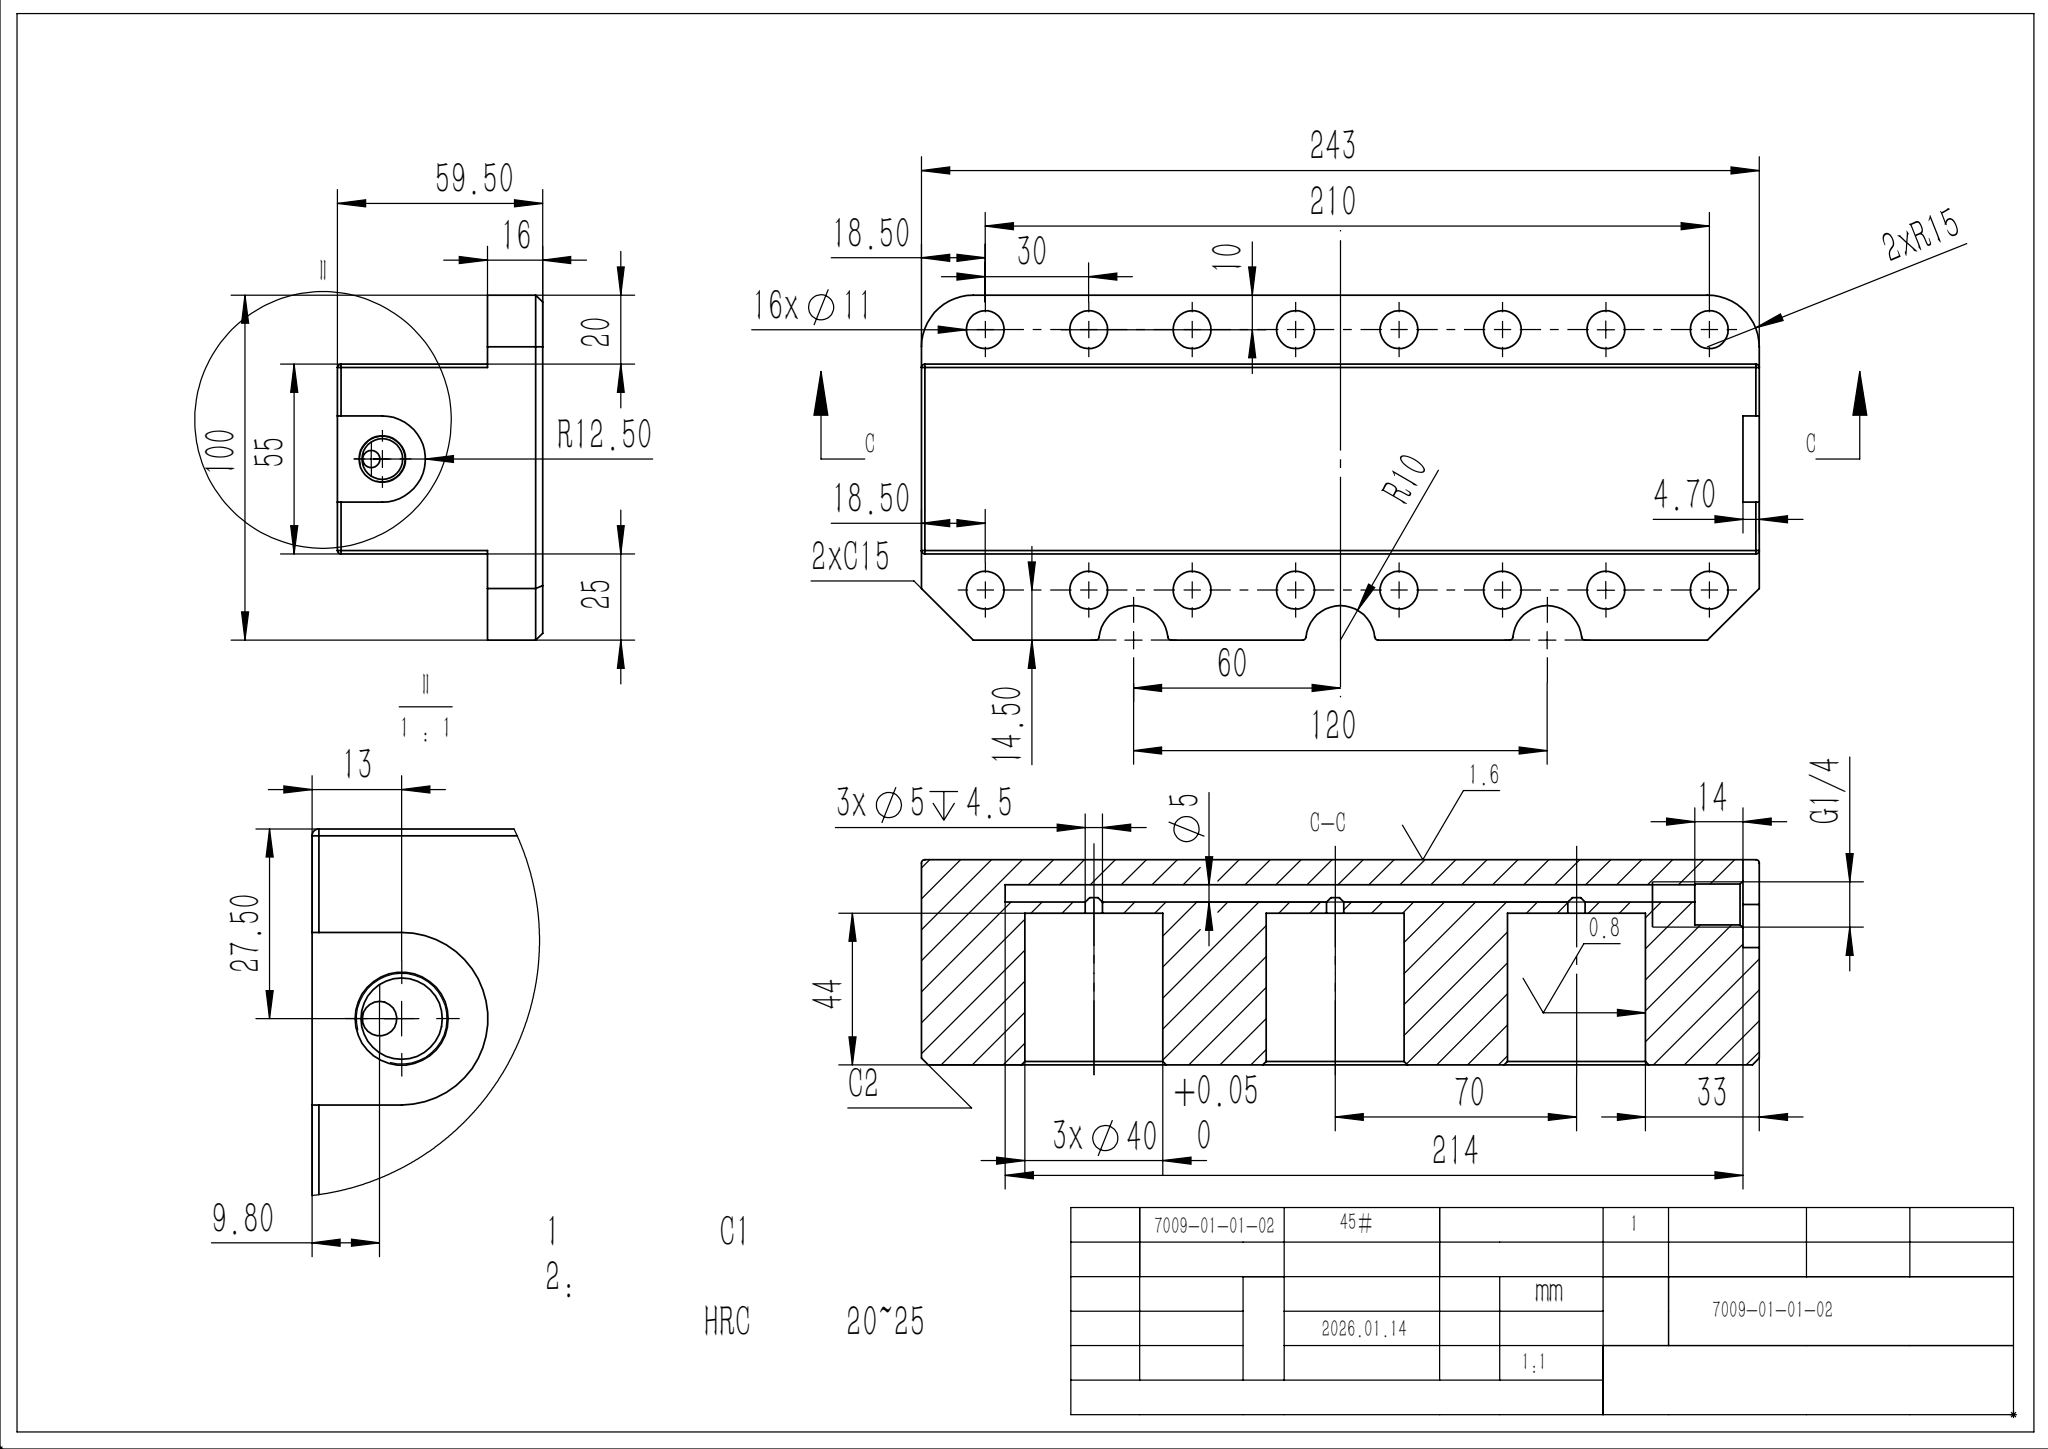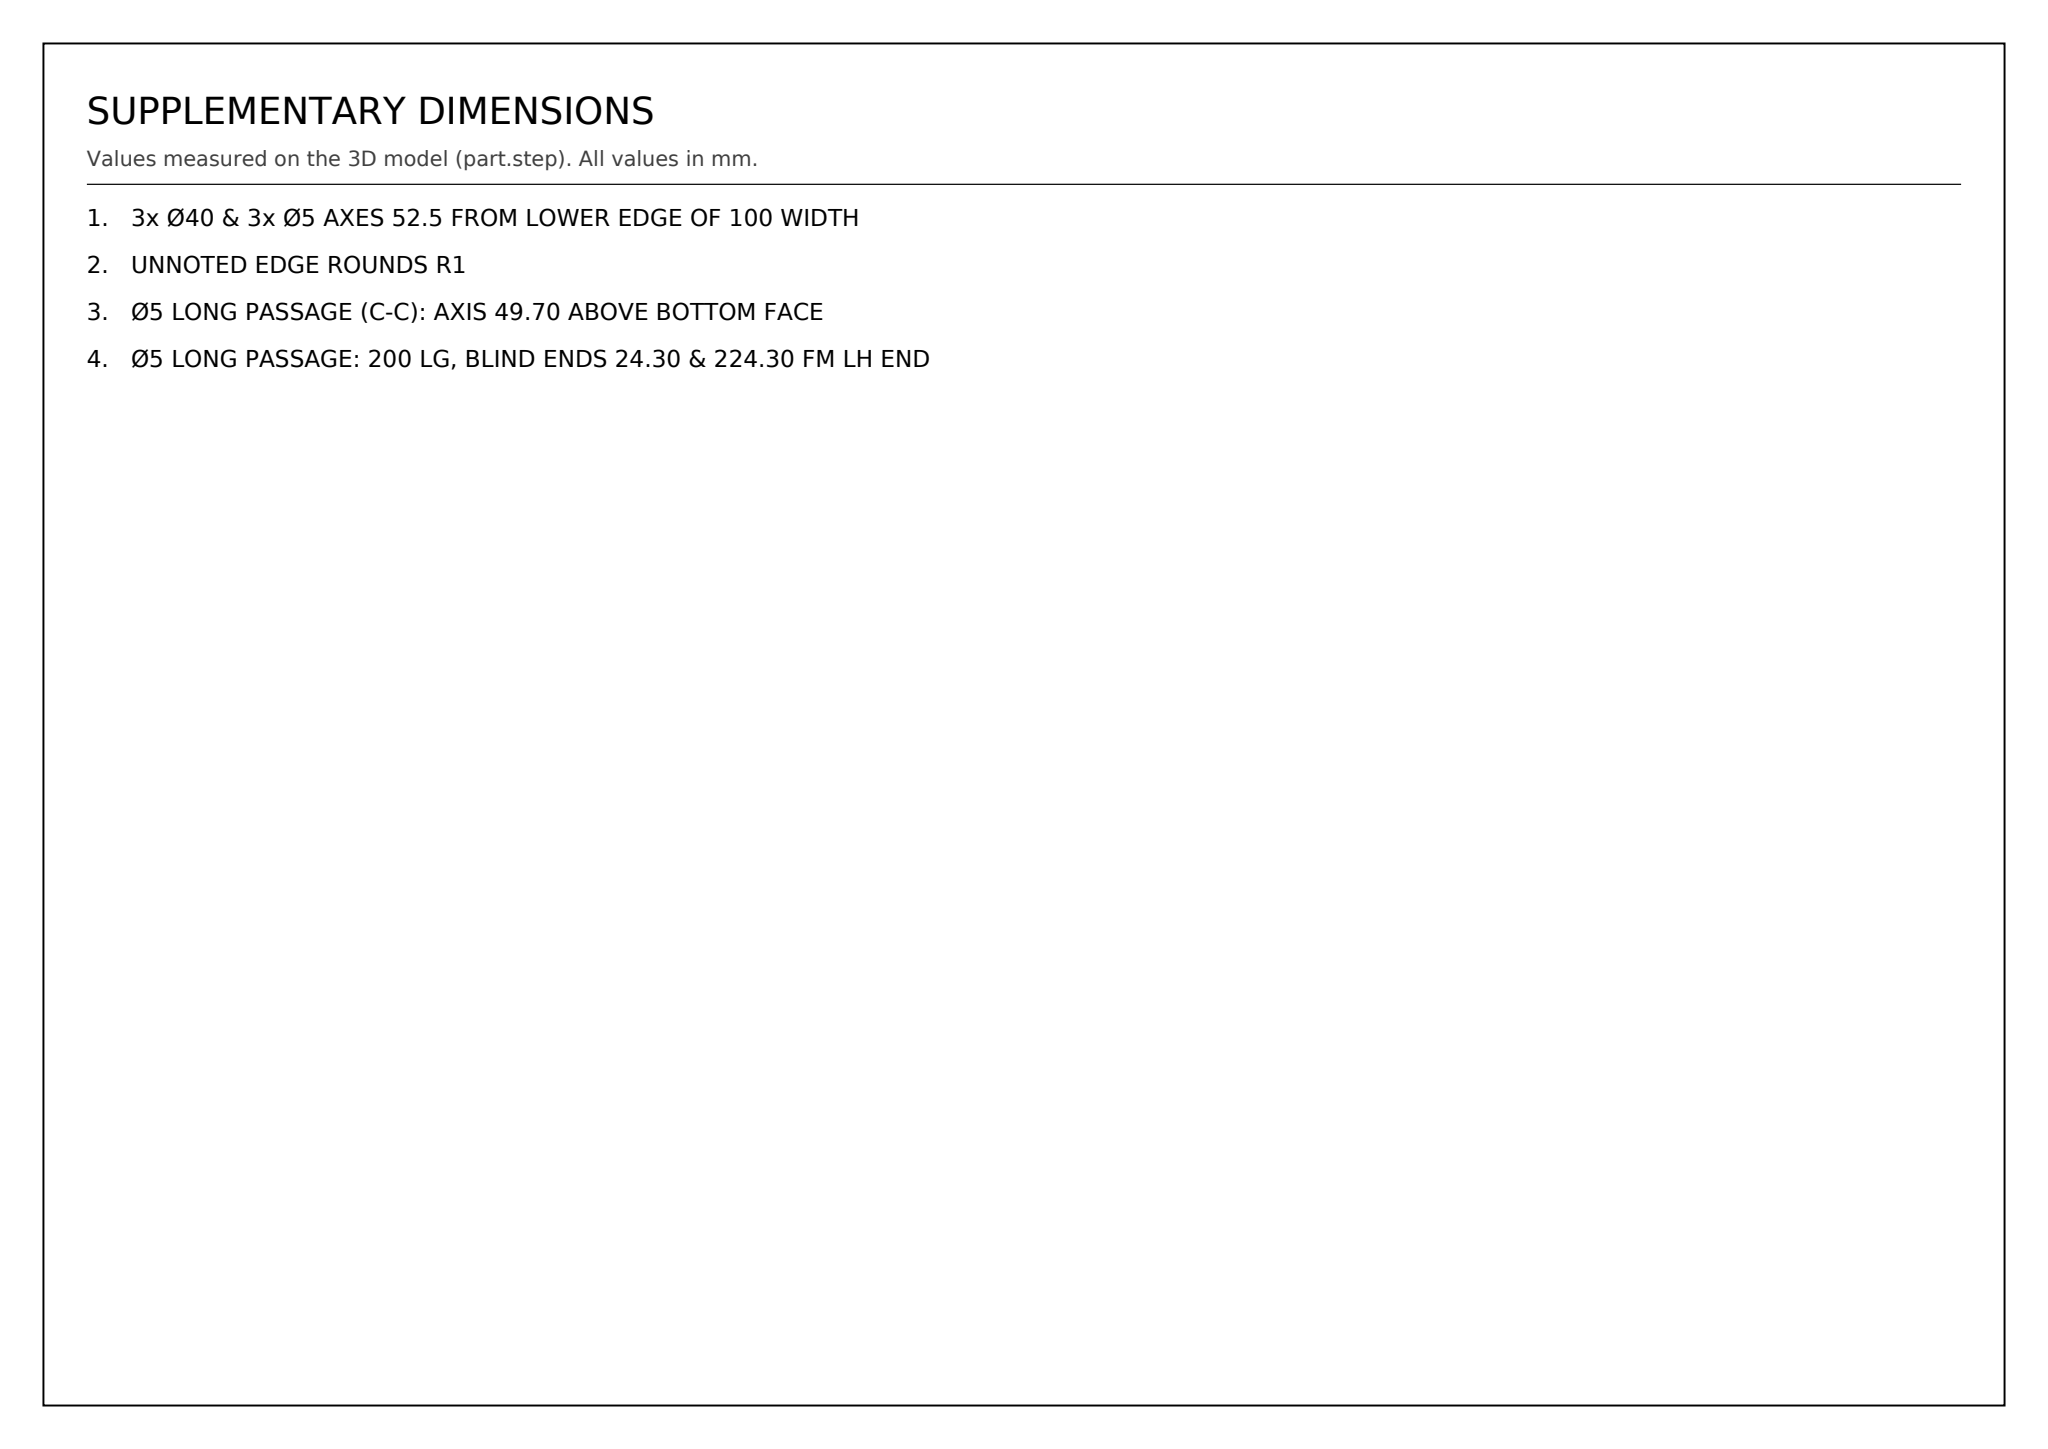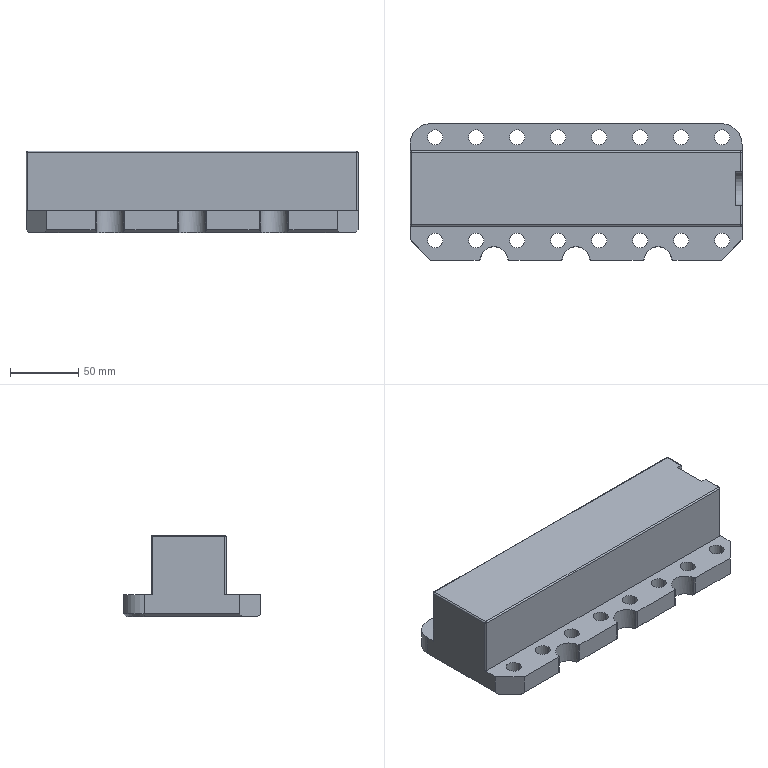Part | SolidWorks | mm | 1 solid | 119 faces | box 243 x 100 x 59.5 mm | volume 757451 mm3 | cylinder 69 | plane 36 | cone 10 | sphere 4 | commonest cylinder face diameters 11 x32 2 x15 5 x8 40 x6 20 x3 11.8 x2 30 x2 25 x1
Drawing notes:
3x Ø40 & 3x Ø5 AXES 52.5 FROM LOWER EDGE OF 100 WIDTH | from the solid: cyl Ø40 z-axis at y=52.5 (x=50,120,190); Ø5 ↧4.5 at same y=52.5; bbox y=100
UNNOTED EDGE ROUNDS R1 | from the solid: Ø2 cylindrical edge surfaces (r=1) along top, ends and scallops; fillet_radii empty
Ø5 LONG PASSAGE (C-C): AXIS 49.70 ABOVE BOTTOM FACE | from the solid: cyl [5.0,"x",[null,52.5,49.7],200.0] - z=49.7 from bbox min (bottom face)
Ø5 LONG PASSAGE: 200 LG, BLIND ENDS 24.30 & 224.30 FM LH END | from the solid: cyl dia5 axis x len 200; axis_planes x=24.3 and x=224.3; bbox x=243